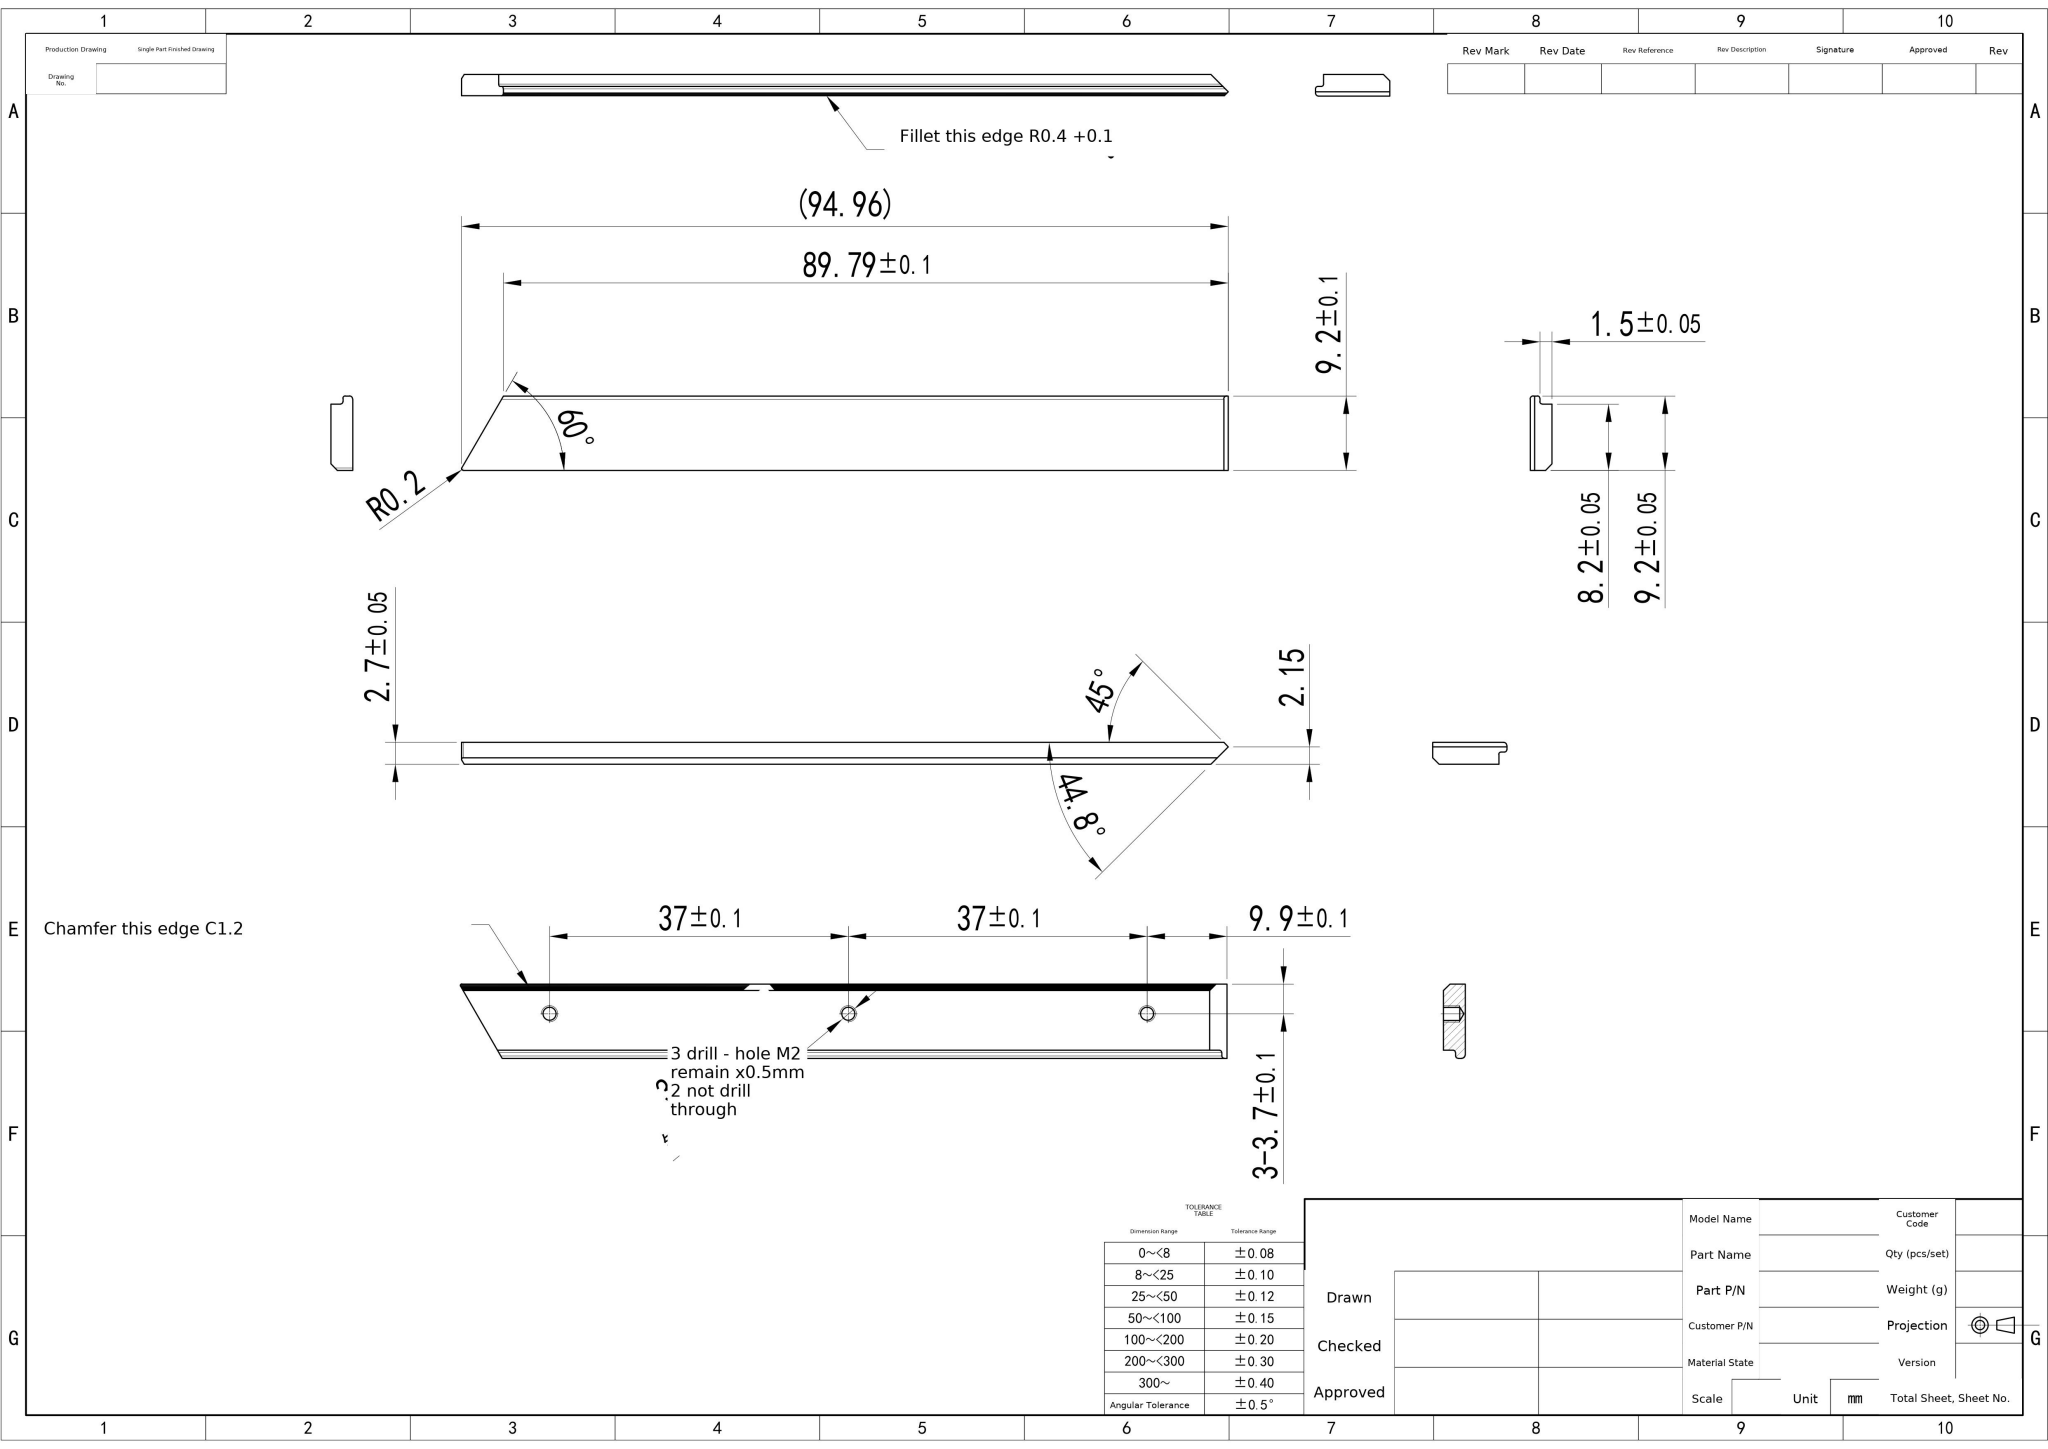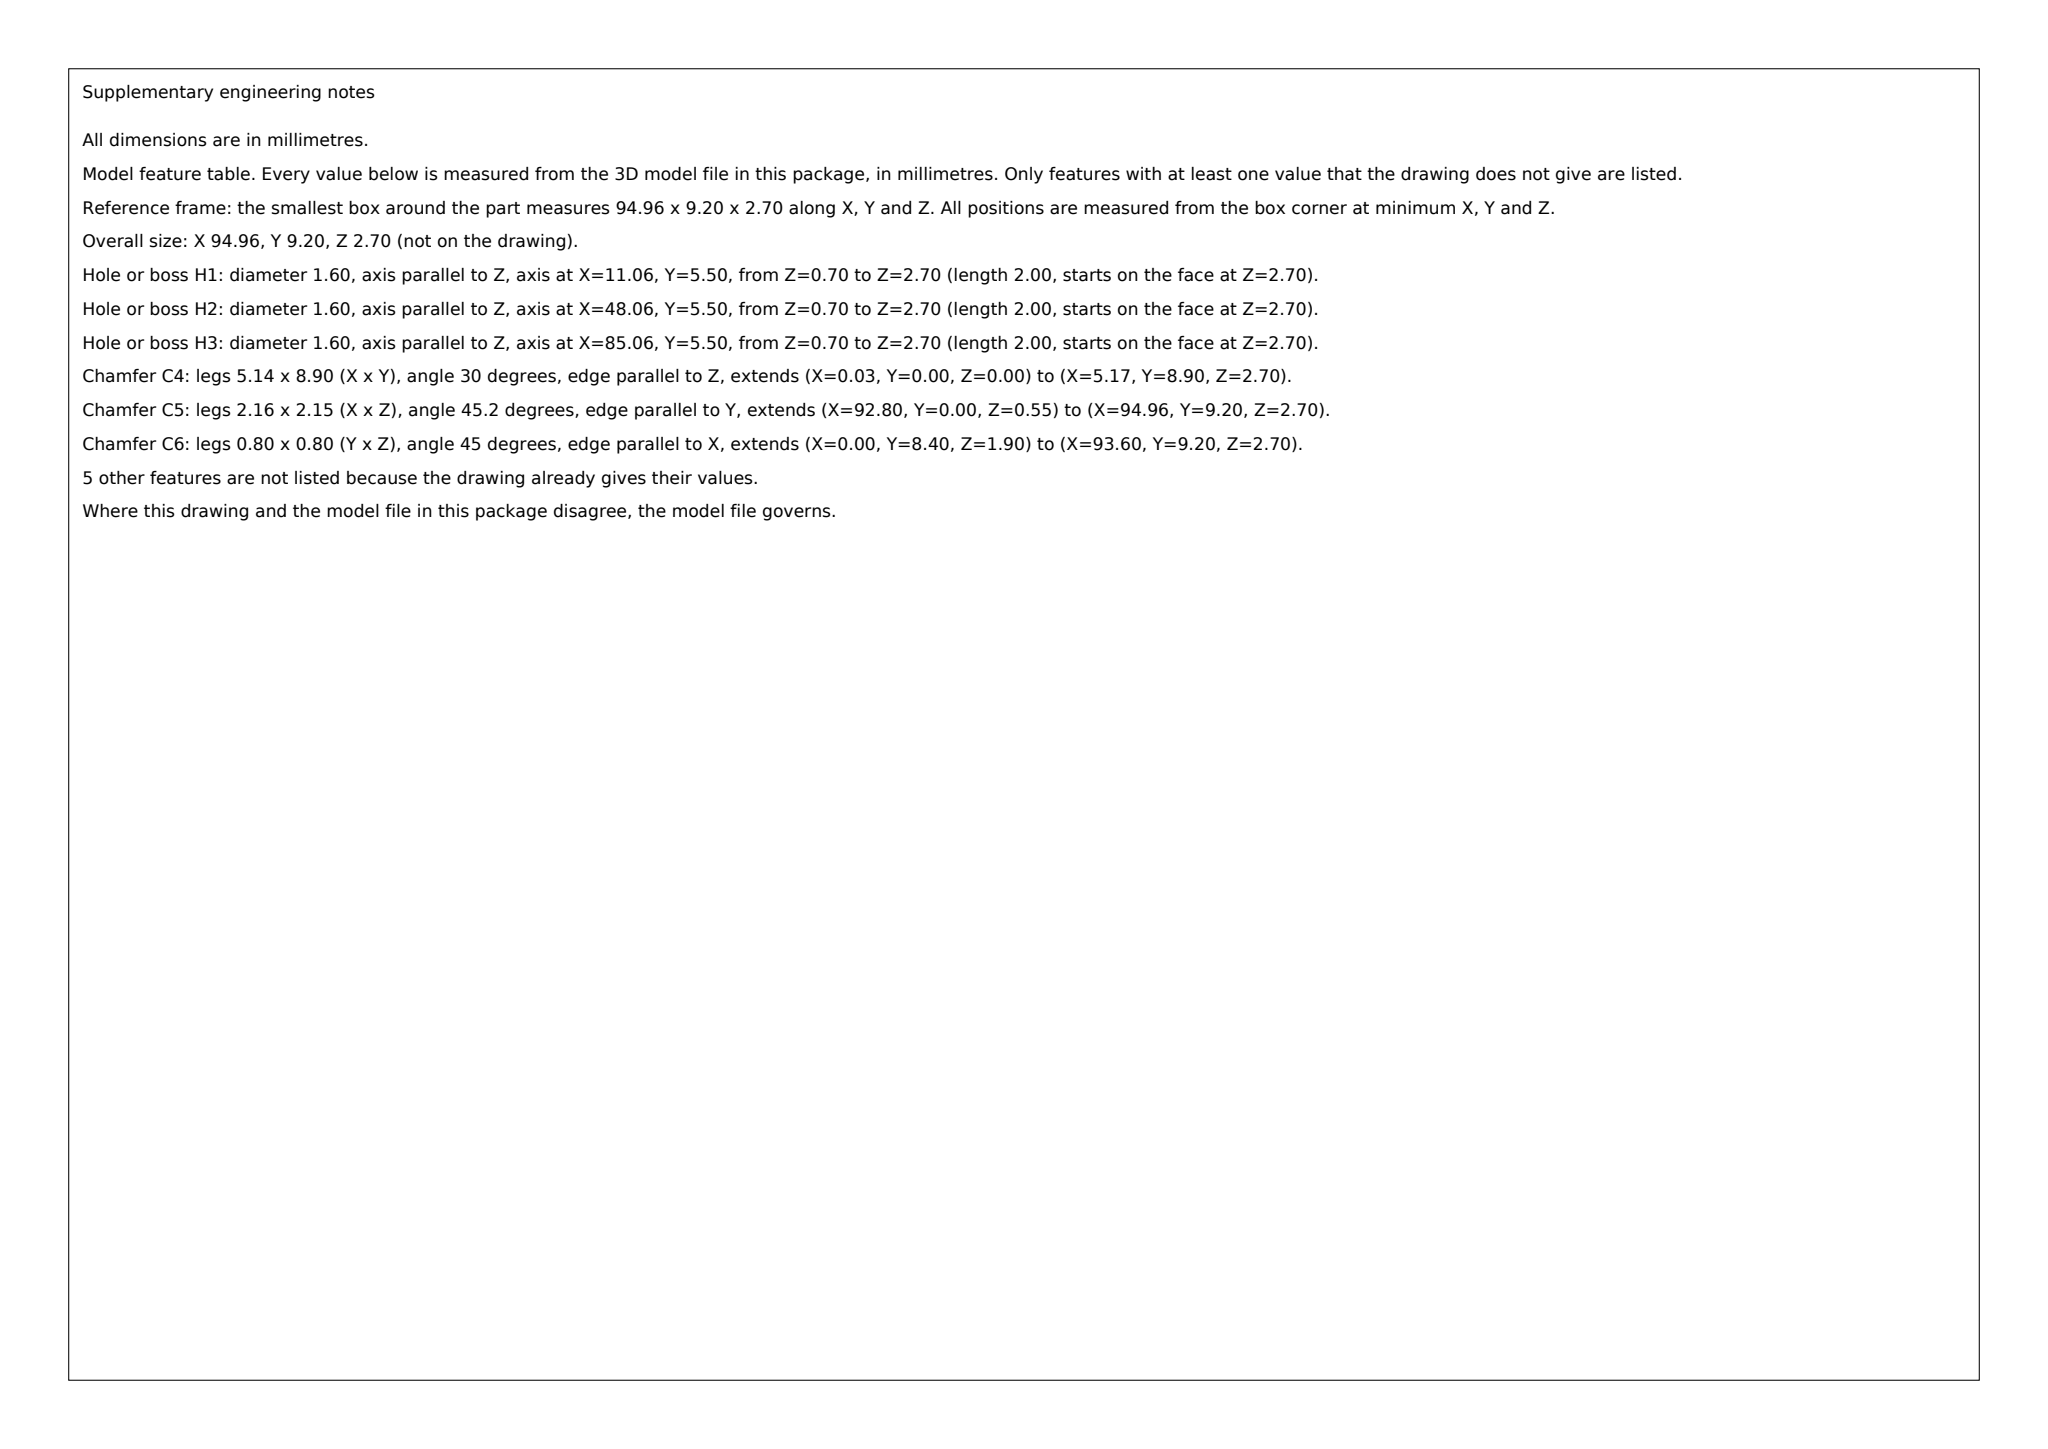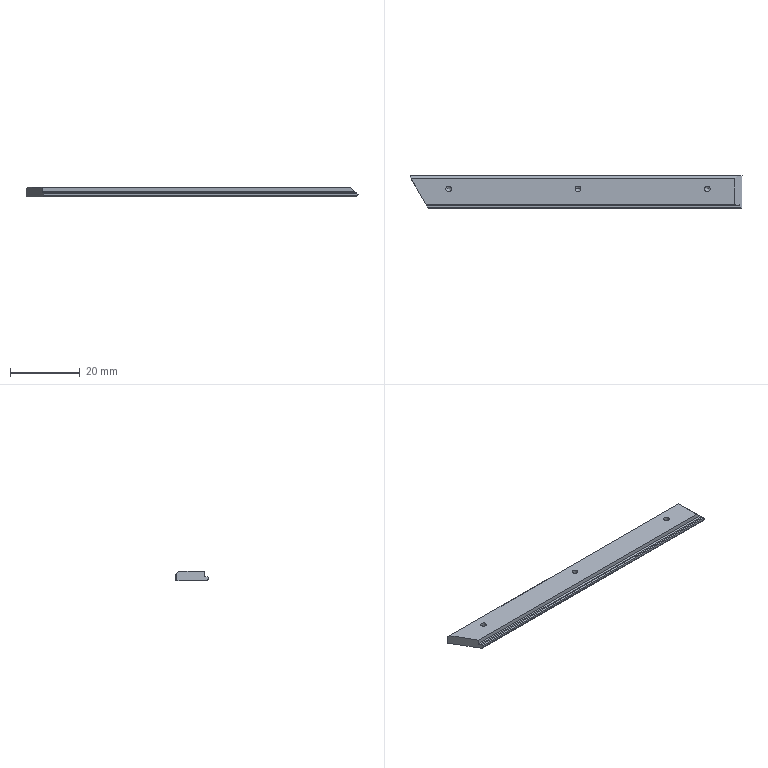Part | SolidWorks | mm | 1 solid | 26 faces | box 94.96 x 9.2 x 2.7 mm | volume 2095 mm3 | cylinder 10 | plane 10 | cone 6 | commonest cylinder face diameters 1.6 x6 0.6 x2 0.8 x1 0.4 x1
STEP:
#1=CARTESIAN_POINT('',(-36.2,0.,0.));
#2=VERTEX_POINT('',#1);
#3=CARTESIAN_POINT('',(-37.8,0.,0.));
#4=VERTEX_POINT('',#3);
#5=CARTESIAN_POINT('',(-37.,0.,0.));
#6=DIRECTION('',(0.,0.,-1.));
#7=DIRECTION('',(-1.,0.,0.));
#8=AXIS2_PLACEMENT_3D('',#5,#6,#7);
#9=CIRCLE('',#8,0.8);
#10=EDGE_CURVE('',#2,#4,#9,.T.);
#11=ORIENTED_EDGE('',*,*,#10,.F.);
#12=CARTESIAN_POINT('',(-36.2,0.,-2.));
#13=VERTEX_POINT('',#12);
#14=CARTESIAN_POINT('',(-36.2,0.,0.));
#15=DIRECTION('',(0.,0.,-1.));
#16=VECTOR('',#15,1000.);
#17=LINE('',#14,#16);
#18=EDGE_CURVE('',#2,#13,#17,.T.);
#19=ORIENTED_EDGE('',*,*,#18,.T.);
#20=CARTESIAN_POINT('',(-37.8,0.,-2.));
#21=VERTEX_POINT('',#20);
#22=CARTESIAN_POINT('',(-37.,0.,-2.));
#23=DIRECTION('',(0.,0.,1.));
#24=DIRECTION('',(-1.,0.,0.));
#25=AXIS2_PLACEMENT_3D('',#22,#23,#24);
#26=CIRCLE('',#25,0.8);
#27=EDGE_CURVE('',#21,#13,#26,.T.);
#28=ORIENTED_EDGE('',*,*,#27,.F.);
#29=CARTESIAN_POINT('',(-37.8,0.,0.));
#30=DIRECTION('',(0.,0.,-1.));
#31=VECTOR('',#30,1000.);
#32=LINE('',#29,#31);
#33=EDGE_CURVE('',#4,#21,#32,.T.);
#34=ORIENTED_EDGE('',*,*,#33,.F.);
#35=EDGE_LOOP('',(#11,#19,#28,#34));
#36=FACE_OUTER_BOUND('',#35,.T.);
#37=CARTESIAN_POINT('',(-37.,0.,0.));
#38=DIRECTION('',(0.,0.,-1.));
#39=DIRECTION('',(-1.,0.,0.));
#40=AXIS2_PLACEMENT_3D('',#37,#38,#39);
#41=CYLINDRICAL_SURFACE('',#40,0.8);
#42=ADVANCED_FACE('',(#36),#41,.F.);
#43=CARTESIAN_POINT('',(0.8,0.,0.));
#44=VERTEX_POINT('',#43);
#45=CARTESIAN_POINT('',(-0.8,0.,0.));
#46=VERTEX_POINT('',#45);
#47=CARTESIAN_POINT('',(0.,0.,0.));
#48=DIRECTION('',(0.,0.,-1.));
#49=DIRECTION('',(-1.,0.,0.));
#50=AXIS2_PLACEMENT_3D('',#47,#48,#49);
#51=CIRCLE('',#50,0.8);
#52=EDGE_CURVE('',#44,#46,#51,.T.);
#53=ORIENTED_EDGE('',*,*,#52,.F.);
#54=CARTESIAN_POINT('',(0.8,0.,-2.));
#55=VERTEX_POINT('',#54);
#56=CARTESIAN_POINT('',(0.8,0.,0.));
#57=DIRECTION('',(0.,0.,-1.));
#58=VECTOR('',#57,1000.);
#59=LINE('',#56,#58);
#60=EDGE_CURVE('',#44,#55,#59,.T.);
#61=ORIENTED_EDGE('',*,*,#60,.T.);
#62=CARTESIAN_POINT('',(-0.8,0.,-2.));
#63=VERTEX_POINT('',#62);
#64=CARTESIAN_POINT('',(0.,0.,-2.));
#65=DIRECTION('',(0.,0.,1.));
#66=DIRECTION('',(-1.,0.,0.));
#67=AXIS2_PLACEMENT_3D('',#64,#65,#66);
#68=CIRCLE('',#67,0.8);
#69=EDGE_CURVE('',#63,#55,#68,.T.);
#70=ORIENTED_EDGE('',*,*,#69,.F.);
#71=CARTESIAN_POINT('',(-0.8,0.,0.));
#72=DIRECTION('',(0.,0.,-1.));
#73=VECTOR('',#72,1000.);
#74=LINE('',#71,#73);
#75=EDGE_CURVE('',#46,#63,#74,.T.);
#76=ORIENTED_EDGE('',*,*,#75,.F.);
#77=EDGE_LOOP('',(#53,#61,#70,#76));
#78=FACE_OUTER_BOUND('',#77,.T.);
#79=CARTESIAN_POINT('',(0.,0.,0.));
#80=DIRECTION('',(0.,0.,-1.));
#81=DIRECTION('',(-1.,0.,0.));
#82=AXIS2_PLACEMENT_3D('',#79,#80,#81);
#83=CYLINDRICAL_SURFACE('',#82,0.8);
#84=ADVANCED_FACE('',(#78),#83,.F.);
#85=CARTESIAN_POINT('',(37.8,0.,0.));
#86=VERTEX_POINT('',#85);
#87=CARTESIAN_POINT('',(36.2,0.,0.));
#88=VERTEX_POINT('',#87);
#89=CARTESIAN_POINT('',(37.,0.,0.));
#90=DIRECTION('',(0.,0.,-1.));
#91=DIRECTION('',(-1.,0.,0.));
#92=AXIS2_PLACEMENT_3D('',#89,#90,#91);
#93=CIRCLE('',#92,0.8);
#94=EDGE_CURVE('',#86,#88,#93,.T.);
#95=ORIENTED_EDGE('',*,*,#94,.F.);
#96=CARTESIAN_POINT('',(37.8,0.,-2.));
#97=VERTEX_POINT('',#96);
#98=CARTESIAN_POINT('',(37.8,0.,0.));
#99=DIRECTION('',(0.,0.,-1.));
#100=VECTOR('',#99,1000.);
#101=LINE('',#98,#100);
#102=EDGE_CURVE('',#86,#97,#101,.T.);
#103=ORIENTED_EDGE('',*,*,#102,.T.);
#104=CARTESIAN_POINT('',(36.2,0.,-2.));
#105=VERTEX_POINT('',#104);
#106=CARTESIAN_POINT('',(37.,0.,-2.));
#107=DIRECTION('',(0.,0.,1.));
#108=DIRECTION('',(-1.,0.,0.));
#109=AXIS2_PLACEMENT_3D('',#106,#107,#108);
#110=CIRCLE('',#109,0.8);
#111=EDGE_CURVE('',#105,#97,#110,.T.);
#112=ORIENTED_EDGE('',*,*,#111,.F.);
#113=CARTESIAN_POINT('',(36.2,0.,0.));
#114=DIRECTION('',(0.,0.,-1.));
#115=VECTOR('',#114,1000.);
#116=LINE('',#113,#115);
#117=EDGE_CURVE('',#88,#105,#116,.T.);
#118=ORIENTED_EDGE('',*,*,#117,.F.);
#119=EDGE_LOOP('',(#95,#103,#112,#118));
#120=FACE_OUTER_BOUND('',#119,.T.);
#121=CARTESIAN_POINT('',(37.,0.,0.));
#122=DIRECTION('',(0.,0.,-1.));
#123=DIRECTION('',(-1.,0.,0.));
#124=AXIS2_PLACEMENT_3D('',#121,#122,#123);
#125=CYLINDRICAL_SURFACE('',#124,0.8);
#126=ADVANCED_FACE('',(#120),#125,.F.);
#127=CARTESIAN_POINT('',(-37.,0.,-2.481));
#128=VERTEX_POINT('',#127);
#129=CARTESIAN_POINT('',(-36.2,0.,-2.));
#130=DIRECTION('',(0.8572,0.,0.515));
#131=VECTOR('',#130,1000.);
#132=LINE('',#129,#131);
#133=EDGE_CURVE('',#128,#13,#132,.T.);
#134=ORIENTED_EDGE('',*,*,#133,.F.);
#135=CARTESIAN_POINT('',(-37.8,0.,-2.));
#136=DIRECTION('',(-0.8572,0.,0.515));
#137=VECTOR('',#136,1000.);
#138=LINE('',#135,#137);
#139=EDGE_CURVE('',#128,#21,#138,.T.);
#140=ORIENTED_EDGE('',*,*,#139,.T.);
#141=ORIENTED_EDGE('',*,*,#27,.T.);
#142=EDGE_LOOP('',(#134,#140,#141));
#143=FACE_OUTER_BOUND('',#142,.T.);
#144=CARTESIAN_POINT('',(-37.,0.,-2.));
#145=DIRECTION('',(0.,0.,1.));
#146=DIRECTION('',(1.,0.,0.));
#147=AXIS2_PLACEMENT_3D('',#144,#145,#146);
#148=CONICAL_SURFACE('',#147,0.8,1.03);
#149=ADVANCED_FACE('',(#143),#148,.F.);
#150=CARTESIAN_POINT('',(0.,0.,-2.481));
#151=VERTEX_POINT('',#150);
#152=CARTESIAN_POINT('',(0.8,0.,-2.));
#153=DIRECTION('',(0.8572,0.,0.515));
#154=VECTOR('',#153,1000.);
#155=LINE('',#152,#154);
#156=EDGE_CURVE('',#151,#55,#155,.T.);
#157=ORIENTED_EDGE('',*,*,#156,.F.);
#158=CARTESIAN_POINT('',(-0.8,0.,-2.));
#159=DIRECTION('',(-0.8572,0.,0.515));
#160=VECTOR('',#159,1000.);
#161=LINE('',#158,#160);
#162=EDGE_CURVE('',#151,#63,#161,.T.);
#163=ORIENTED_EDGE('',*,*,#162,.T.);
#164=ORIENTED_EDGE('',*,*,#69,.T.);
#165=EDGE_LOOP('',(#157,#163,#164));
#166=FACE_OUTER_BOUND('',#165,.T.);
#167=CARTESIAN_POINT('',(0.,0.,-2.));
#168=DIRECTION('',(0.,0.,1.));
#169=DIRECTION('',(1.,0.,0.));
#170=AXIS2_PLACEMENT_3D('',#167,#168,#169);
#171=CONICAL_SURFACE('',#170,0.8,1.03);
#172=ADVANCED_FACE('',(#166),#171,.F.);
#173=CARTESIAN_POINT('',(37.,0.,-2.481));
#174=VERTEX_POINT('',#173);
#175=CARTESIAN_POINT('',(37.8,0.,-2.));
#176=DIRECTION('',(0.8572,0.,0.515));
#177=VECTOR('',#176,1000.);
#178=LINE('',#175,#177);
#179=EDGE_CURVE('',#174,#97,#178,.T.);
#180=ORIENTED_EDGE('',*,*,#179,.F.);
#181=CARTESIAN_POINT('',(36.2,0.,-2.));
#182=DIRECTION('',(-0.8572,0.,0.515));
#183=VECTOR('',#182,1000.);
#184=LINE('',#181,#183);
#185=EDGE_CURVE('',#174,#105,#184,.T.);
#186=ORIENTED_EDGE('',*,*,#185,.T.);
#187=ORIENTED_EDGE('',*,*,#111,.T.);
#188=EDGE_LOOP('',(#180,#186,#187));
#189=FACE_OUTER_BOUND('',#188,.T.);
#190=CARTESIAN_POINT('',(37.,0.,-2.));
#191=DIRECTION('',(0.,0.,1.));
#192=DIRECTION('',(1.,0.,0.));
#193=AXIS2_PLACEMENT_3D('',#190,#191,#192);
#194=CONICAL_SURFACE('',#193,0.8,1.03);
#195=ADVANCED_FACE('',(#189),#194,.F.);
#196=CARTESIAN_POINT('',(-47.86,3.7,-2.7));
#197=VERTEX_POINT('',#196);
#198=CARTESIAN_POINT('',(-48.033,3.4,-2.7));
#199=VERTEX_POINT('',#198);
#200=CARTESIAN_POINT('',(-47.86,3.5,-2.7));
#201=DIRECTION('',(0.,0.,1.));
#202=DIRECTION('',(1.,0.,0.));
#203=AXIS2_PLACEMENT_3D('',#200,#201,#202);
#204=CIRCLE('',#203,0.2);
#205=EDGE_CURVE('',#197,#199,#204,.T.);
#206=ORIENTED_EDGE('',*,*,#205,.F.);
#207=CARTESIAN_POINT('',(46.349,3.7,-2.7));
#208=VERTEX_POINT('',#207);
#209=CARTESIAN_POINT('',(-253.1,3.7,-2.7));
#210=DIRECTION('',(1.,0.,0.));
#211=VECTOR('',#210,1000.);
#212=LINE('',#209,#211);
#213=EDGE_CURVE('',#197,#208,#212,.T.);
#214=ORIENTED_EDGE('',*,*,#213,.T.);
#215=CARTESIAN_POINT('',(46.349,-5.1,-2.7));
#216=VERTEX_POINT('',#215);
#217=CARTESIAN_POINT('',(46.349,-5.1,-2.7));
#218=DIRECTION('',(0.,-1.,0.));
#219=VECTOR('',#218,1000.);
#220=LINE('',#217,#219);
#221=EDGE_CURVE('',#208,#216,#220,.T.);
#222=ORIENTED_EDGE('',*,*,#221,.T.);
#223=CARTESIAN_POINT('',(-43.125,-5.1,-2.7));
#224=VERTEX_POINT('',#223);
#225=CARTESIAN_POINT('',(-253.1,-5.1,-2.7));
#226=DIRECTION('',(-1.,0.,0.));
#227=VECTOR('',#226,1000.);
#228=LINE('',#225,#227);
#229=EDGE_CURVE('',#216,#224,#228,.T.);
#230=ORIENTED_EDGE('',*,*,#229,.T.);
#231=CARTESIAN_POINT('',(-43.125,-5.1,-2.7));
#232=DIRECTION('',(-0.5,0.866,0.));
#233=VECTOR('',#232,1000.);
#234=LINE('',#231,#233);
#235=EDGE_CURVE('',#224,#199,#234,.T.);
#236=ORIENTED_EDGE('',*,*,#235,.T.);
#237=EDGE_LOOP('',(#206,#214,#222,#230,#236));
#238=FACE_OUTER_BOUND('',#237,.T.);
#239=CARTESIAN_POINT('',(-253.1,-5.1,-2.7));
#240=DIRECTION('',(0.,0.,-1.));
#241=DIRECTION('',(-1.,0.,0.));
#242=AXIS2_PLACEMENT_3D('',#239,#240,#241);
#243=PLANE('',#242);
#244=ADVANCED_FACE('',(#238),#243,.T.);
#245=CARTESIAN_POINT('',(-47.86,3.7,-0.8));
#246=VERTEX_POINT('',#245);
#247=CARTESIAN_POINT('',(-47.86,3.7,-2.7));
#248=DIRECTION('',(0.,0.,1.));
#249=VECTOR('',#248,1000.);
#250=LINE('',#247,#249);
#251=EDGE_CURVE('',#197,#246,#250,.T.);
#252=ORIENTED_EDGE('',*,*,#251,.T.);
#253=CARTESIAN_POINT('',(45.542,3.7,-0.8));
#254=VERTEX_POINT('',#253);
#255=CARTESIAN_POINT('',(-253.1,3.7,-0.8));
#256=DIRECTION('',(1.,0.,0.));
#257=VECTOR('',#256,1000.);
#258=LINE('',#255,#257);
#259=EDGE_CURVE('',#246,#254,#258,.T.);
#260=ORIENTED_EDGE('',*,*,#259,.T.);
#261=CARTESIAN_POINT('',(46.9,3.7,-2.149));
#262=VERTEX_POINT('',#261);
#263=CARTESIAN_POINT('',(45.542,3.7,-0.8));
#264=DIRECTION('',(0.7096,0.,-0.7046));
#265=VECTOR('',#264,1000.);
#266=LINE('',#263,#265);
#267=EDGE_CURVE('',#254,#262,#266,.T.);
#268=ORIENTED_EDGE('',*,*,#267,.T.);
#269=CARTESIAN_POINT('',(46.9,3.7,-2.149));
#270=DIRECTION('',(-0.7071,0.,-0.7071));
#271=VECTOR('',#270,1000.);
#272=LINE('',#269,#271);
#273=EDGE_CURVE('',#262,#208,#272,.T.);
#274=ORIENTED_EDGE('',*,*,#273,.T.);
#275=ORIENTED_EDGE('',*,*,#213,.F.);
#276=EDGE_LOOP('',(#252,#260,#268,#274,#275));
#277=FACE_OUTER_BOUND('',#276,.T.);
#278=CARTESIAN_POINT('',(-253.1,3.7,-2.7));
#279=DIRECTION('',(0.,1.,0.));
#280=DIRECTION('',(0.,0.,1.));
#281=AXIS2_PLACEMENT_3D('',#278,#279,#280);
#282=PLANE('',#281);
#283=ADVANCED_FACE('',(#277),#282,.T.);
#284=CARTESIAN_POINT('',(-43.472,-4.5,-0.));
#285=VERTEX_POINT('',#284);
#286=CARTESIAN_POINT('',(-43.472,-4.5,-1.2));
#287=VERTEX_POINT('',#286);
#288=CARTESIAN_POINT('',(-43.472,-4.5,-0.));
#289=DIRECTION('',(0.,0.,-1.));
#290=VECTOR('',#289,1000.);
#291=LINE('',#288,#290);
#292=EDGE_CURVE('',#285,#287,#291,.T.);
#293=ORIENTED_EDGE('',*,*,#292,.F.);
#294=CARTESIAN_POINT('',(-47.744,2.9,-0.));
#295=VERTEX_POINT('',#294);
#296=CARTESIAN_POINT('',(-48.033,3.4,-0.));
#297=DIRECTION('',(-0.5,0.866,0.));
#298=VECTOR('',#297,1000.);
#299=LINE('',#296,#298);
#300=EDGE_CURVE('',#285,#295,#299,.T.);
#301=ORIENTED_EDGE('',*,*,#300,.T.);
#302=CARTESIAN_POINT('',(-48.033,3.4,-0.5));
#303=VERTEX_POINT('',#302);
#304=CARTESIAN_POINT('',(-47.744,2.9,-0.));
#305=DIRECTION('',(-0.378,0.6547,-0.6547));
#306=VECTOR('',#305,1000.);
#307=LINE('',#304,#306);
#308=EDGE_CURVE('',#295,#303,#307,.T.);
#309=ORIENTED_EDGE('',*,*,#308,.T.);
#310=CARTESIAN_POINT('',(-48.033,3.4,-300.));
#311=DIRECTION('',(0.,0.,-1.));
#312=VECTOR('',#311,1000.);
#313=LINE('',#310,#312);
#314=EDGE_CURVE('',#303,#199,#313,.T.);
#315=ORIENTED_EDGE('',*,*,#314,.T.);
#316=ORIENTED_EDGE('',*,*,#235,.F.);
#317=CARTESIAN_POINT('',(-42.894,-5.5,-2.3));
#318=VERTEX_POINT('',#317);
#319=CARTESIAN_POINT('',(-43.125,-5.1,-2.7));
#320=CARTESIAN_POINT('',(-42.99,-5.334,-2.7));
#321=CARTESIAN_POINT('',(-42.894,-5.5,-2.534));
#322=CARTESIAN_POINT('',(-42.894,-5.5,-2.3));
#323=(BOUNDED_CURVE()B_SPLINE_CURVE(3,(#319,#320,#321,#322),.UNSPECIFIED.,.F.,.T.)B_SPLINE_CURVE_WITH_KNOTS((4,4),(4.712,6.283),.UNSPECIFIED.)CURVE()GEOMETRIC_REPRESENTATION_ITEM()RATIONAL_B_SPLINE_CURVE((1.,0.8047,0.8047,1.))REPRESENTATION_ITEM(''));
#324=EDGE_CURVE('',#224,#318,#323,.T.);
#325=ORIENTED_EDGE('',*,*,#324,.T.);
#326=CARTESIAN_POINT('',(-42.894,-5.5,-1.8));
#327=VERTEX_POINT('',#326);
#328=CARTESIAN_POINT('',(-42.894,-5.5,-1.8));
#329=DIRECTION('',(0.,0.,-1.));
#330=VECTOR('',#329,1000.);
#331=LINE('',#328,#330);
#332=EDGE_CURVE('',#327,#318,#331,.T.);
#333=ORIENTED_EDGE('',*,*,#332,.F.);
#334=CARTESIAN_POINT('',(-43.068,-5.2,-1.5));
#335=VERTEX_POINT('',#334);
#336=CARTESIAN_POINT('',(-43.068,-5.2,-1.5));
#337=CARTESIAN_POINT('',(-42.966,-5.376,-1.5));
#338=CARTESIAN_POINT('',(-42.894,-5.5,-1.624));
#339=CARTESIAN_POINT('',(-42.894,-5.5,-1.8));
#340=(BOUNDED_CURVE()B_SPLINE_CURVE(3,(#336,#337,#338,#339),.UNSPECIFIED.,.F.,.F.)B_SPLINE_CURVE_WITH_KNOTS((4,4),(4.712,6.283),.UNSPECIFIED.)CURVE()GEOMETRIC_REPRESENTATION_ITEM()RATIONAL_B_SPLINE_CURVE((1.,0.8047,0.8047,1.))REPRESENTATION_ITEM(''));
#341=EDGE_CURVE('',#335,#327,#340,.T.);
#342=ORIENTED_EDGE('',*,*,#341,.F.);
#343=CARTESIAN_POINT('',(-43.299,-4.8,-1.5));
#344=VERTEX_POINT('',#343);
#345=CARTESIAN_POINT('',(-43.299,-4.8,-1.5));
#346=DIRECTION('',(0.5,-0.866,0.));
#347=VECTOR('',#346,1000.);
#348=LINE('',#345,#347);
#349=EDGE_CURVE('',#344,#335,#348,.T.);
#350=ORIENTED_EDGE('',*,*,#349,.F.);
#351=CARTESIAN_POINT('',(-43.299,-4.8,-1.5));
#352=CARTESIAN_POINT('',(-43.4,-4.624,-1.5));
#353=CARTESIAN_POINT('',(-43.472,-4.5,-1.376));
#354=CARTESIAN_POINT('',(-43.472,-4.5,-1.2));
#355=(BOUNDED_CURVE()B_SPLINE_CURVE(3,(#351,#352,#353,#354),.UNSPECIFIED.,.F.,.F.)B_SPLINE_CURVE_WITH_KNOTS((4,4),(1.571,3.142),.UNSPECIFIED.)CURVE()GEOMETRIC_REPRESENTATION_ITEM()RATIONAL_B_SPLINE_CURVE((1.,0.8047,0.8047,1.))REPRESENTATION_ITEM(''));
#356=EDGE_CURVE('',#344,#287,#355,.T.);
#357=ORIENTED_EDGE('',*,*,#356,.T.);
#358=EDGE_LOOP('',(#293,#301,#309,#315,#316,#325,#333,#342,#350,#357));
#359=FACE_OUTER_BOUND('',#358,.T.);
#360=CARTESIAN_POINT('',(-48.033,3.4,-300.));
#361=DIRECTION('',(-0.866,-0.5,0.));
#362=DIRECTION('',(0.5,-0.866,0.));
#363=AXIS2_PLACEMENT_3D('',#360,#361,#362);
#364=PLANE('',#363);
#365=ADVANCED_FACE('',(#359),#364,.T.);
#366=ORIENTED_EDGE('',*,*,#324,.F.);
#367=ORIENTED_EDGE('',*,*,#229,.F.);
#368=CARTESIAN_POINT('',(46.749,-5.5,-2.3));
#369=VERTEX_POINT('',#368);
#370=CARTESIAN_POINT('',(46.349,-5.1,-2.7));
#371=CARTESIAN_POINT('',(46.349,-5.334,-2.7));
#372=CARTESIAN_POINT('',(46.514,-5.5,-2.534));
#373=CARTESIAN_POINT('',(46.749,-5.5,-2.3));
#374=(BOUNDED_CURVE()B_SPLINE_CURVE(3,(#370,#371,#372,#373),.UNSPECIFIED.,.F.,.F.)B_SPLINE_CURVE_WITH_KNOTS((4,4),(3.142,4.712),.UNSPECIFIED.)CURVE()GEOMETRIC_REPRESENTATION_ITEM()RATIONAL_B_SPLINE_CURVE((1.,0.8047,0.8047,1.))REPRESENTATION_ITEM(''));
#375=EDGE_CURVE('',#216,#369,#374,.T.);
#376=ORIENTED_EDGE('',*,*,#375,.T.);
#377=CARTESIAN_POINT('',(-253.1,-5.5,-2.3));
#378=DIRECTION('',(-1.,0.,0.));
#379=VECTOR('',#378,1000.);
#380=LINE('',#377,#379);
#381=EDGE_CURVE('',#369,#318,#380,.T.);
#382=ORIENTED_EDGE('',*,*,#381,.T.);
#383=EDGE_LOOP('',(#366,#367,#376,#382));
#384=FACE_OUTER_BOUND('',#383,.T.);
#385=CARTESIAN_POINT('',(-253.1,-5.1,-2.3));
#386=DIRECTION('',(1.,0.,0.));
#387=DIRECTION('',(0.,0.,-1.));
#388=AXIS2_PLACEMENT_3D('',#385,#386,#387);
#389=CYLINDRICAL_SURFACE('',#388,0.4);
#390=ADVANCED_FACE('',(#384),#389,.T.);
#391=CARTESIAN_POINT('',(46.9,-5.5,-2.149));
#392=VERTEX_POINT('',#391);
#393=CARTESIAN_POINT('',(46.349,-5.5,-2.7));
#394=DIRECTION('',(0.7071,0.,0.7071));
#395=VECTOR('',#394,1000.);
#396=LINE('',#393,#395);
#397=EDGE_CURVE('',#369,#392,#396,.T.);
#398=ORIENTED_EDGE('',*,*,#397,.F.);
#399=ORIENTED_EDGE('',*,*,#375,.F.);
#400=ORIENTED_EDGE('',*,*,#221,.F.);
#401=ORIENTED_EDGE('',*,*,#273,.F.);
#402=CARTESIAN_POINT('',(46.9,-296.3,-2.149));
#403=DIRECTION('',(0.,1.,0.));
#404=VECTOR('',#403,1000.);
#405=LINE('',#402,#404);
#406=EDGE_CURVE('',#392,#262,#405,.T.);
#407=ORIENTED_EDGE('',*,*,#406,.F.);
#408=EDGE_LOOP('',(#398,#399,#400,#401,#407));
#409=FACE_OUTER_BOUND('',#408,.T.);
#410=CARTESIAN_POINT('',(46.349,-296.3,-2.7));
#411=DIRECTION('',(-0.7071,0.,0.7071));
#412=DIRECTION('',(0.7071,0.,0.7071));
#413=AXIS2_PLACEMENT_3D('',#410,#411,#412);
#414=PLANE('',#413);
#415=ADVANCED_FACE('',(#409),#414,.F.);
#416=ORIENTED_EDGE('',*,*,#308,.F.);
#417=CARTESIAN_POINT('',(44.736,2.9,-0.));
#418=VERTEX_POINT('',#417);
#419=CARTESIAN_POINT('',(-253.1,2.9,-0.));
#420=DIRECTION('',(1.,0.,0.));
#421=VECTOR('',#420,1000.);
#422=LINE('',#419,#421);
#423=EDGE_CURVE('',#295,#418,#422,.T.);
#424=ORIENTED_EDGE('',*,*,#423,.T.);
#425=CARTESIAN_POINT('',(44.736,2.9,-0.));
#426=DIRECTION('',(0.58,0.576,-0.576));
#427=VECTOR('',#426,1000.);
#428=LINE('',#425,#427);
#429=EDGE_CURVE('',#418,#254,#428,.T.);
#430=ORIENTED_EDGE('',*,*,#429,.T.);
#431=ORIENTED_EDGE('',*,*,#259,.F.);
#432=CARTESIAN_POINT('',(-47.86,3.7,-0.8));
#433=CARTESIAN_POINT('',(-48.033,3.7,-0.8));
#434=CARTESIAN_POINT('',(-48.119,3.55,-0.65));
#435=CARTESIAN_POINT('',(-48.033,3.4,-0.5));
#436=(BOUNDED_CURVE()B_SPLINE_CURVE(3,(#432,#433,#434,#435),.UNSPECIFIED.,.F.,.T.)B_SPLINE_CURVE_WITH_KNOTS((4,4),(3.142,5.236),.UNSPECIFIED.)CURVE()GEOMETRIC_REPRESENTATION_ITEM()RATIONAL_B_SPLINE_CURVE((1.,0.6667,0.6667,1.))REPRESENTATION_ITEM(''));
#437=EDGE_CURVE('',#246,#303,#436,.T.);
#438=ORIENTED_EDGE('',*,*,#437,.T.);
#439=EDGE_LOOP('',(#416,#424,#430,#431,#438));
#440=FACE_OUTER_BOUND('',#439,.T.);
#441=CARTESIAN_POINT('',(-253.1,3.7,-0.8));
#442=DIRECTION('',(0.,0.7071,0.7071));
#443=DIRECTION('',(0.,-0.7071,0.7071));
#444=AXIS2_PLACEMENT_3D('',#441,#442,#443);
#445=PLANE('',#444);
#446=ADVANCED_FACE('',(#440),#445,.T.);
#447=ORIENTED_EDGE('',*,*,#251,.F.);
#448=ORIENTED_EDGE('',*,*,#205,.T.);
#449=ORIENTED_EDGE('',*,*,#314,.F.);
#450=ORIENTED_EDGE('',*,*,#437,.F.);
#451=EDGE_LOOP('',(#447,#448,#449,#450));
#452=FACE_OUTER_BOUND('',#451,.T.);
#453=CARTESIAN_POINT('',(-47.86,3.5,-300.));
#454=DIRECTION('',(0.,0.,1.));
#455=DIRECTION('',(1.,0.,0.));
#456=AXIS2_PLACEMENT_3D('',#453,#454,#455);
#457=CYLINDRICAL_SURFACE('',#456,0.2);
#458=ADVANCED_FACE('',(#452),#457,.T.);
#459=ORIENTED_EDGE('',*,*,#429,.F.);
#460=CARTESIAN_POINT('',(44.736,-4.5,-0.));
#461=VERTEX_POINT('',#460);
#462=CARTESIAN_POINT('',(44.736,-296.3,-0.));
#463=DIRECTION('',(0.,1.,0.));
#464=VECTOR('',#463,1000.);
#465=LINE('',#462,#464);
#466=EDGE_CURVE('',#461,#418,#465,.T.);
#467=ORIENTED_EDGE('',*,*,#466,.F.);
#468=CARTESIAN_POINT('',(45.945,-4.5,-1.2));
#469=VERTEX_POINT('',#468);
#470=CARTESIAN_POINT('',(45.945,-4.5,-1.2));
#471=DIRECTION('',(-0.7096,0.,0.7046));
#472=VECTOR('',#471,1000.);
#473=LINE('',#470,#472);
#474=EDGE_CURVE('',#469,#461,#473,.T.);
#475=ORIENTED_EDGE('',*,*,#474,.F.);
#476=CARTESIAN_POINT('',(46.247,-4.8,-1.5));
#477=VERTEX_POINT('',#476);
#478=CARTESIAN_POINT('',(45.945,-4.5,-1.2));
#479=CARTESIAN_POINT('',(46.122,-4.5,-1.376));
#480=CARTESIAN_POINT('',(46.247,-4.624,-1.5));
#481=CARTESIAN_POINT('',(46.247,-4.8,-1.5));
#482=(BOUNDED_CURVE()B_SPLINE_CURVE(3,(#478,#479,#480,#481),.UNSPECIFIED.,.F.,.F.)B_SPLINE_CURVE_WITH_KNOTS((4,4),(4.712,6.283),.UNSPECIFIED.)CURVE()GEOMETRIC_REPRESENTATION_ITEM()RATIONAL_B_SPLINE_CURVE((1.,0.8047,0.8047,1.))REPRESENTATION_ITEM(''));
#483=EDGE_CURVE('',#469,#477,#482,.T.);
#484=ORIENTED_EDGE('',*,*,#483,.T.);
#485=CARTESIAN_POINT('',(46.247,-5.2,-1.5));
#486=VERTEX_POINT('',#485);
#487=CARTESIAN_POINT('',(46.247,-4.8,-1.5));
#488=DIRECTION('',(0.,1.,0.));
#489=VECTOR('',#488,1000.);
#490=LINE('',#487,#489);
#491=EDGE_CURVE('',#486,#477,#490,.T.);
#492=ORIENTED_EDGE('',*,*,#491,.F.);
#493=CARTESIAN_POINT('',(46.549,-5.5,-1.8));
#494=VERTEX_POINT('',#493);
#495=CARTESIAN_POINT('',(46.549,-5.5,-1.8));
#496=CARTESIAN_POINT('',(46.372,-5.5,-1.624));
#497=CARTESIAN_POINT('',(46.247,-5.376,-1.5));
#498=CARTESIAN_POINT('',(46.247,-5.2,-1.5));
#499=(BOUNDED_CURVE()B_SPLINE_CURVE(3,(#495,#496,#497,#498),.UNSPECIFIED.,.F.,.F.)B_SPLINE_CURVE_WITH_KNOTS((4,4),(1.571,3.142),.UNSPECIFIED.)CURVE()GEOMETRIC_REPRESENTATION_ITEM()RATIONAL_B_SPLINE_CURVE((1.,0.8047,0.8047,1.))REPRESENTATION_ITEM(''));
#500=EDGE_CURVE('',#494,#486,#499,.T.);
#501=ORIENTED_EDGE('',*,*,#500,.F.);
#502=CARTESIAN_POINT('',(46.9,-5.5,-2.149));
#503=DIRECTION('',(-0.7096,0.,0.7046));
#504=VECTOR('',#503,1000.);
#505=LINE('',#502,#504);
#506=EDGE_CURVE('',#392,#494,#505,.T.);
#507=ORIENTED_EDGE('',*,*,#506,.F.);
#508=ORIENTED_EDGE('',*,*,#406,.T.);
#509=ORIENTED_EDGE('',*,*,#267,.F.);
#510=EDGE_LOOP('',(#459,#467,#475,#484,#492,#501,#507,#508,#509));
#511=FACE_OUTER_BOUND('',#510,.T.);
#512=CARTESIAN_POINT('',(46.9,-296.3,-2.149));
#513=DIRECTION('',(-0.7046,0.,-0.7096));
#514=DIRECTION('',(-0.7096,0.,0.7046));
#515=AXIS2_PLACEMENT_3D('',#512,#513,#514);
#516=PLANE('',#515);
#517=ADVANCED_FACE('',(#511),#516,.F.);
#518=ORIENTED_EDGE('',*,*,#423,.F.);
#519=ORIENTED_EDGE('',*,*,#300,.F.);
#520=CARTESIAN_POINT('',(-253.1,-4.5,-0.));
#521=DIRECTION('',(1.,0.,0.));
#522=VECTOR('',#521,1000.);
#523=LINE('',#520,#522);
#524=EDGE_CURVE('',#285,#461,#523,.T.);
#525=ORIENTED_EDGE('',*,*,#524,.T.);
#526=ORIENTED_EDGE('',*,*,#466,.T.);
#527=EDGE_LOOP('',(#518,#519,#525,#526));
#528=FACE_OUTER_BOUND('',#527,.T.);
#529=CARTESIAN_POINT('',(-37.,0.,0.));
#530=DIRECTION('',(0.,0.,-1.));
#531=DIRECTION('',(-1.,0.,0.));
#532=AXIS2_PLACEMENT_3D('',#529,#530,#531);
#533=CIRCLE('',#532,0.8);
#534=EDGE_CURVE('',#4,#2,#533,.T.);
#535=ORIENTED_EDGE('',*,*,#534,.T.);
#536=ORIENTED_EDGE('',*,*,#10,.T.);
#537=EDGE_LOOP('',(#535,#536));
#538=FACE_BOUND('',#537,.T.);
#539=CARTESIAN_POINT('',(0.,0.,0.));
#540=DIRECTION('',(0.,0.,-1.));
#541=DIRECTION('',(-1.,0.,0.));
#542=AXIS2_PLACEMENT_3D('',#539,#540,#541);
#543=CIRCLE('',#542,0.8);
#544=EDGE_CURVE('',#46,#44,#543,.T.);
#545=ORIENTED_EDGE('',*,*,#544,.T.);
#546=ORIENTED_EDGE('',*,*,#52,.T.);
#547=EDGE_LOOP('',(#545,#546));
#548=FACE_BOUND('',#547,.T.);
#549=CARTESIAN_POINT('',(37.,0.,0.));
#550=DIRECTION('',(0.,0.,-1.));
#551=DIRECTION('',(-1.,0.,0.));
#552=AXIS2_PLACEMENT_3D('',#549,#550,#551);
#553=CIRCLE('',#552,0.8);
#554=EDGE_CURVE('',#88,#86,#553,.T.);
#555=ORIENTED_EDGE('',*,*,#554,.T.);
#556=ORIENTED_EDGE('',*,*,#94,.T.);
#557=EDGE_LOOP('',(#555,#556));
#558=FACE_BOUND('',#557,.T.);
#559=CARTESIAN_POINT('',(-253.1,2.9,-0.));
#560=DIRECTION('',(0.,0.,1.));
#561=DIRECTION('',(1.,0.,0.));
#562=AXIS2_PLACEMENT_3D('',#559,#560,#561);
#563=PLANE('',#562);
#564=ADVANCED_FACE('',(#528,#538,#548,#558),#563,.T.);
#565=ORIENTED_EDGE('',*,*,#332,.T.);
#566=ORIENTED_EDGE('',*,*,#381,.F.);
#567=ORIENTED_EDGE('',*,*,#397,.T.);
#568=ORIENTED_EDGE('',*,*,#506,.T.);
#569=CARTESIAN_POINT('',(-253.1,-5.5,-1.8));
#570=DIRECTION('',(-1.,0.,0.));
#571=VECTOR('',#570,1000.);
#572=LINE('',#569,#571);
#573=EDGE_CURVE('',#494,#327,#572,.T.);
#574=ORIENTED_EDGE('',*,*,#573,.T.);
#575=EDGE_LOOP('',(#565,#566,#567,#568,#574));
#576=FACE_OUTER_BOUND('',#575,.T.);
#577=CARTESIAN_POINT('',(-253.1,-5.5,-1.8));
#578=DIRECTION('',(0.,-1.,0.));
#579=DIRECTION('',(0.,0.,-1.));
#580=AXIS2_PLACEMENT_3D('',#577,#578,#579);
#581=PLANE('',#580);
#582=ADVANCED_FACE('',(#576),#581,.T.);
#583=ORIENTED_EDGE('',*,*,#292,.T.);
#584=CARTESIAN_POINT('',(-253.1,-4.5,-1.2));
#585=DIRECTION('',(1.,0.,0.));
#586=VECTOR('',#585,1000.);
#587=LINE('',#584,#586);
#588=EDGE_CURVE('',#287,#469,#587,.T.);
#589=ORIENTED_EDGE('',*,*,#588,.T.);
#590=ORIENTED_EDGE('',*,*,#474,.T.);
#591=ORIENTED_EDGE('',*,*,#524,.F.);
#592=EDGE_LOOP('',(#583,#589,#590,#591));
#593=FACE_OUTER_BOUND('',#592,.T.);
#594=CARTESIAN_POINT('',(-253.1,-4.5,-0.));
#595=DIRECTION('',(0.,-1.,0.));
#596=DIRECTION('',(0.,0.,-1.));
#597=AXIS2_PLACEMENT_3D('',#594,#595,#596);
#598=PLANE('',#597);
#599=ADVANCED_FACE('',(#593),#598,.T.);
#600=ORIENTED_EDGE('',*,*,#18,.F.);
#601=ORIENTED_EDGE('',*,*,#534,.F.);
#602=ORIENTED_EDGE('',*,*,#33,.T.);
#603=CARTESIAN_POINT('',(-37.,0.,-2.));
#604=DIRECTION('',(0.,0.,1.));
#605=DIRECTION('',(-1.,0.,0.));
#606=AXIS2_PLACEMENT_3D('',#603,#604,#605);
#607=CIRCLE('',#606,0.8);
#608=EDGE_CURVE('',#13,#21,#607,.T.);
#609=ORIENTED_EDGE('',*,*,#608,.F.);
#610=EDGE_LOOP('',(#600,#601,#602,#609));
#611=FACE_OUTER_BOUND('',#610,.T.);
#612=CARTESIAN_POINT('',(-37.,0.,0.));
#613=DIRECTION('',(0.,0.,-1.));
#614=DIRECTION('',(-1.,0.,0.));
#615=AXIS2_PLACEMENT_3D('',#612,#613,#614);
#616=CYLINDRICAL_SURFACE('',#615,0.8);
#617=ADVANCED_FACE('',(#611),#616,.F.);
#618=ORIENTED_EDGE('',*,*,#60,.F.);
#619=ORIENTED_EDGE('',*,*,#544,.F.);
#620=ORIENTED_EDGE('',*,*,#75,.T.);
#621=CARTESIAN_POINT('',(0.,0.,-2.));
#622=DIRECTION('',(0.,0.,1.));
#623=DIRECTION('',(-1.,0.,0.));
#624=AXIS2_PLACEMENT_3D('',#621,#622,#623);
#625=CIRCLE('',#624,0.8);
#626=EDGE_CURVE('',#55,#63,#625,.T.);
#627=ORIENTED_EDGE('',*,*,#626,.F.);
#628=EDGE_LOOP('',(#618,#619,#620,#627));
#629=FACE_OUTER_BOUND('',#628,.T.);
#630=CARTESIAN_POINT('',(0.,0.,0.));
#631=DIRECTION('',(0.,0.,-1.));
#632=DIRECTION('',(-1.,0.,0.));
#633=AXIS2_PLACEMENT_3D('',#630,#631,#632);
#634=CYLINDRICAL_SURFACE('',#633,0.8);
#635=ADVANCED_FACE('',(#629),#634,.F.);
#636=ORIENTED_EDGE('',*,*,#102,.F.);
#637=ORIENTED_EDGE('',*,*,#554,.F.);
#638=ORIENTED_EDGE('',*,*,#117,.T.);
#639=CARTESIAN_POINT('',(37.,0.,-2.));
#640=DIRECTION('',(0.,0.,1.));
#641=DIRECTION('',(-1.,0.,0.));
#642=AXIS2_PLACEMENT_3D('',#639,#640,#641);
#643=CIRCLE('',#642,0.8);
#644=EDGE_CURVE('',#97,#105,#643,.T.);
#645=ORIENTED_EDGE('',*,*,#644,.F.);
#646=EDGE_LOOP('',(#636,#637,#638,#645));
#647=FACE_OUTER_BOUND('',#646,.T.);
#648=CARTESIAN_POINT('',(37.,0.,0.));
#649=DIRECTION('',(0.,0.,-1.));
#650=DIRECTION('',(-1.,0.,0.));
#651=AXIS2_PLACEMENT_3D('',#648,#649,#650);
#652=CYLINDRICAL_SURFACE('',#651,0.8);
#653=ADVANCED_FACE('',(#647),#652,.F.);
#654=ORIENTED_EDGE('',*,*,#341,.T.);
#655=ORIENTED_EDGE('',*,*,#573,.F.);
#656=ORIENTED_EDGE('',*,*,#500,.T.);
#657=CARTESIAN_POINT('',(-253.1,-5.2,-1.5));
#658=DIRECTION('',(-1.,0.,0.));
#659=VECTOR('',#658,1000.);
#660=LINE('',#657,#659);
#661=EDGE_CURVE('',#486,#335,#660,.T.);
#662=ORIENTED_EDGE('',*,*,#661,.T.);
#663=EDGE_LOOP('',(#654,#655,#656,#662));
#664=FACE_OUTER_BOUND('',#663,.T.);
#665=CARTESIAN_POINT('',(-253.1,-5.2,-1.8));
#666=DIRECTION('',(1.,0.,0.));
#667=DIRECTION('',(0.,0.,-1.));
#668=AXIS2_PLACEMENT_3D('',#665,#666,#667);
#669=CYLINDRICAL_SURFACE('',#668,0.3);
#670=ADVANCED_FACE('',(#664),#669,.T.);
#671=ORIENTED_EDGE('',*,*,#588,.F.);
#672=ORIENTED_EDGE('',*,*,#356,.F.);
#673=CARTESIAN_POINT('',(-253.1,-4.8,-1.5));
#674=DIRECTION('',(-1.,0.,0.));
#675=VECTOR('',#674,1000.);
#676=LINE('',#673,#675);
#677=EDGE_CURVE('',#477,#344,#676,.T.);
#678=ORIENTED_EDGE('',*,*,#677,.F.);
#679=ORIENTED_EDGE('',*,*,#483,.F.);
#680=EDGE_LOOP('',(#671,#672,#678,#679));
#681=FACE_OUTER_BOUND('',#680,.T.);
#682=CARTESIAN_POINT('',(-253.1,-4.8,-1.2));
#683=DIRECTION('',(1.,0.,0.));
#684=DIRECTION('',(0.,0.,-1.));
#685=AXIS2_PLACEMENT_3D('',#682,#683,#684);
#686=CYLINDRICAL_SURFACE('',#685,0.3);
#687=ADVANCED_FACE('',(#681),#686,.F.);
#688=ORIENTED_EDGE('',*,*,#139,.F.);
#689=ORIENTED_EDGE('',*,*,#133,.T.);
#690=ORIENTED_EDGE('',*,*,#608,.T.);
#691=EDGE_LOOP('',(#688,#689,#690));
#692=FACE_OUTER_BOUND('',#691,.T.);
#693=CARTESIAN_POINT('',(-37.,0.,-2.));
#694=DIRECTION('',(0.,0.,1.));
#695=DIRECTION('',(1.,0.,0.));
#696=AXIS2_PLACEMENT_3D('',#693,#694,#695);
#697=CONICAL_SURFACE('',#696,0.8,1.03);
#698=ADVANCED_FACE('',(#692),#697,.F.);
#699=ORIENTED_EDGE('',*,*,#162,.F.);
#700=ORIENTED_EDGE('',*,*,#156,.T.);
#701=ORIENTED_EDGE('',*,*,#626,.T.);
#702=EDGE_LOOP('',(#699,#700,#701));
#703=FACE_OUTER_BOUND('',#702,.T.);
#704=CARTESIAN_POINT('',(0.,0.,-2.));
#705=DIRECTION('',(0.,0.,1.));
#706=DIRECTION('',(1.,0.,0.));
#707=AXIS2_PLACEMENT_3D('',#704,#705,#706);
#708=CONICAL_SURFACE('',#707,0.8,1.03);
#709=ADVANCED_FACE('',(#703),#708,.F.);
#710=ORIENTED_EDGE('',*,*,#185,.F.);
#711=ORIENTED_EDGE('',*,*,#179,.T.);
#712=ORIENTED_EDGE('',*,*,#644,.T.);
#713=EDGE_LOOP('',(#710,#711,#712));
#714=FACE_OUTER_BOUND('',#713,.T.);
#715=CARTESIAN_POINT('',(37.,0.,-2.));
#716=DIRECTION('',(0.,0.,1.));
#717=DIRECTION('',(1.,0.,0.));
#718=AXIS2_PLACEMENT_3D('',#715,#716,#717);
#719=CONICAL_SURFACE('',#718,0.8,1.03);
#720=ADVANCED_FACE('',(#714),#719,.F.);
#721=ORIENTED_EDGE('',*,*,#349,.T.);
#722=ORIENTED_EDGE('',*,*,#661,.F.);
#723=ORIENTED_EDGE('',*,*,#491,.T.);
#724=ORIENTED_EDGE('',*,*,#677,.T.);
#725=EDGE_LOOP('',(#721,#722,#723,#724));
#726=FACE_OUTER_BOUND('',#725,.T.);
#727=CARTESIAN_POINT('',(-253.1,-4.8,-1.5));
#728=DIRECTION('',(0.,0.,1.));
#729=DIRECTION('',(1.,0.,0.));
#730=AXIS2_PLACEMENT_3D('',#727,#728,#729);
#731=PLANE('',#730);
#732=ADVANCED_FACE('',(#726),#731,.T.);
#733=CLOSED_SHELL('',(#42,#84,#126,#149,#172,#195,#244,#283,#365,#390,#415,#446,#458,#517,#564,#582,#599,#617,#635,#653,#670,#687,#698,#709,#720,#732));
#734=MANIFOLD_SOLID_BREP('',#733);
#735=CARTESIAN_POINT('',(0.,0.,0.));
#736=DIRECTION('',(0.,0.,1.));
#737=DIRECTION('',(1.,0.,0.));
#738=AXIS2_PLACEMENT_3D('',#735,#736,#737);
#739=(LENGTH_UNIT()NAMED_UNIT(*)SI_UNIT(.MILLI.,.METRE.));
#740=UNCERTAINTY_MEASURE_WITH_UNIT(LENGTH_MEASURE(0.00001),#739,'','');
#741=(NAMED_UNIT(*)PLANE_ANGLE_UNIT()SI_UNIT($,.RADIAN.));
#742=(NAMED_UNIT(*)SI_UNIT($,.STERADIAN.)SOLID_ANGLE_UNIT());
#743=(GEOMETRIC_REPRESENTATION_CONTEXT(3)GLOBAL_UNCERTAINTY_ASSIGNED_CONTEXT((#740))GLOBAL_UNIT_ASSIGNED_CONTEXT((#739,#741,#742))REPRESENTATION_CONTEXT('',''));
#744=ADVANCED_BREP_SHAPE_REPRESENTATION('',(#734,#738),#743);